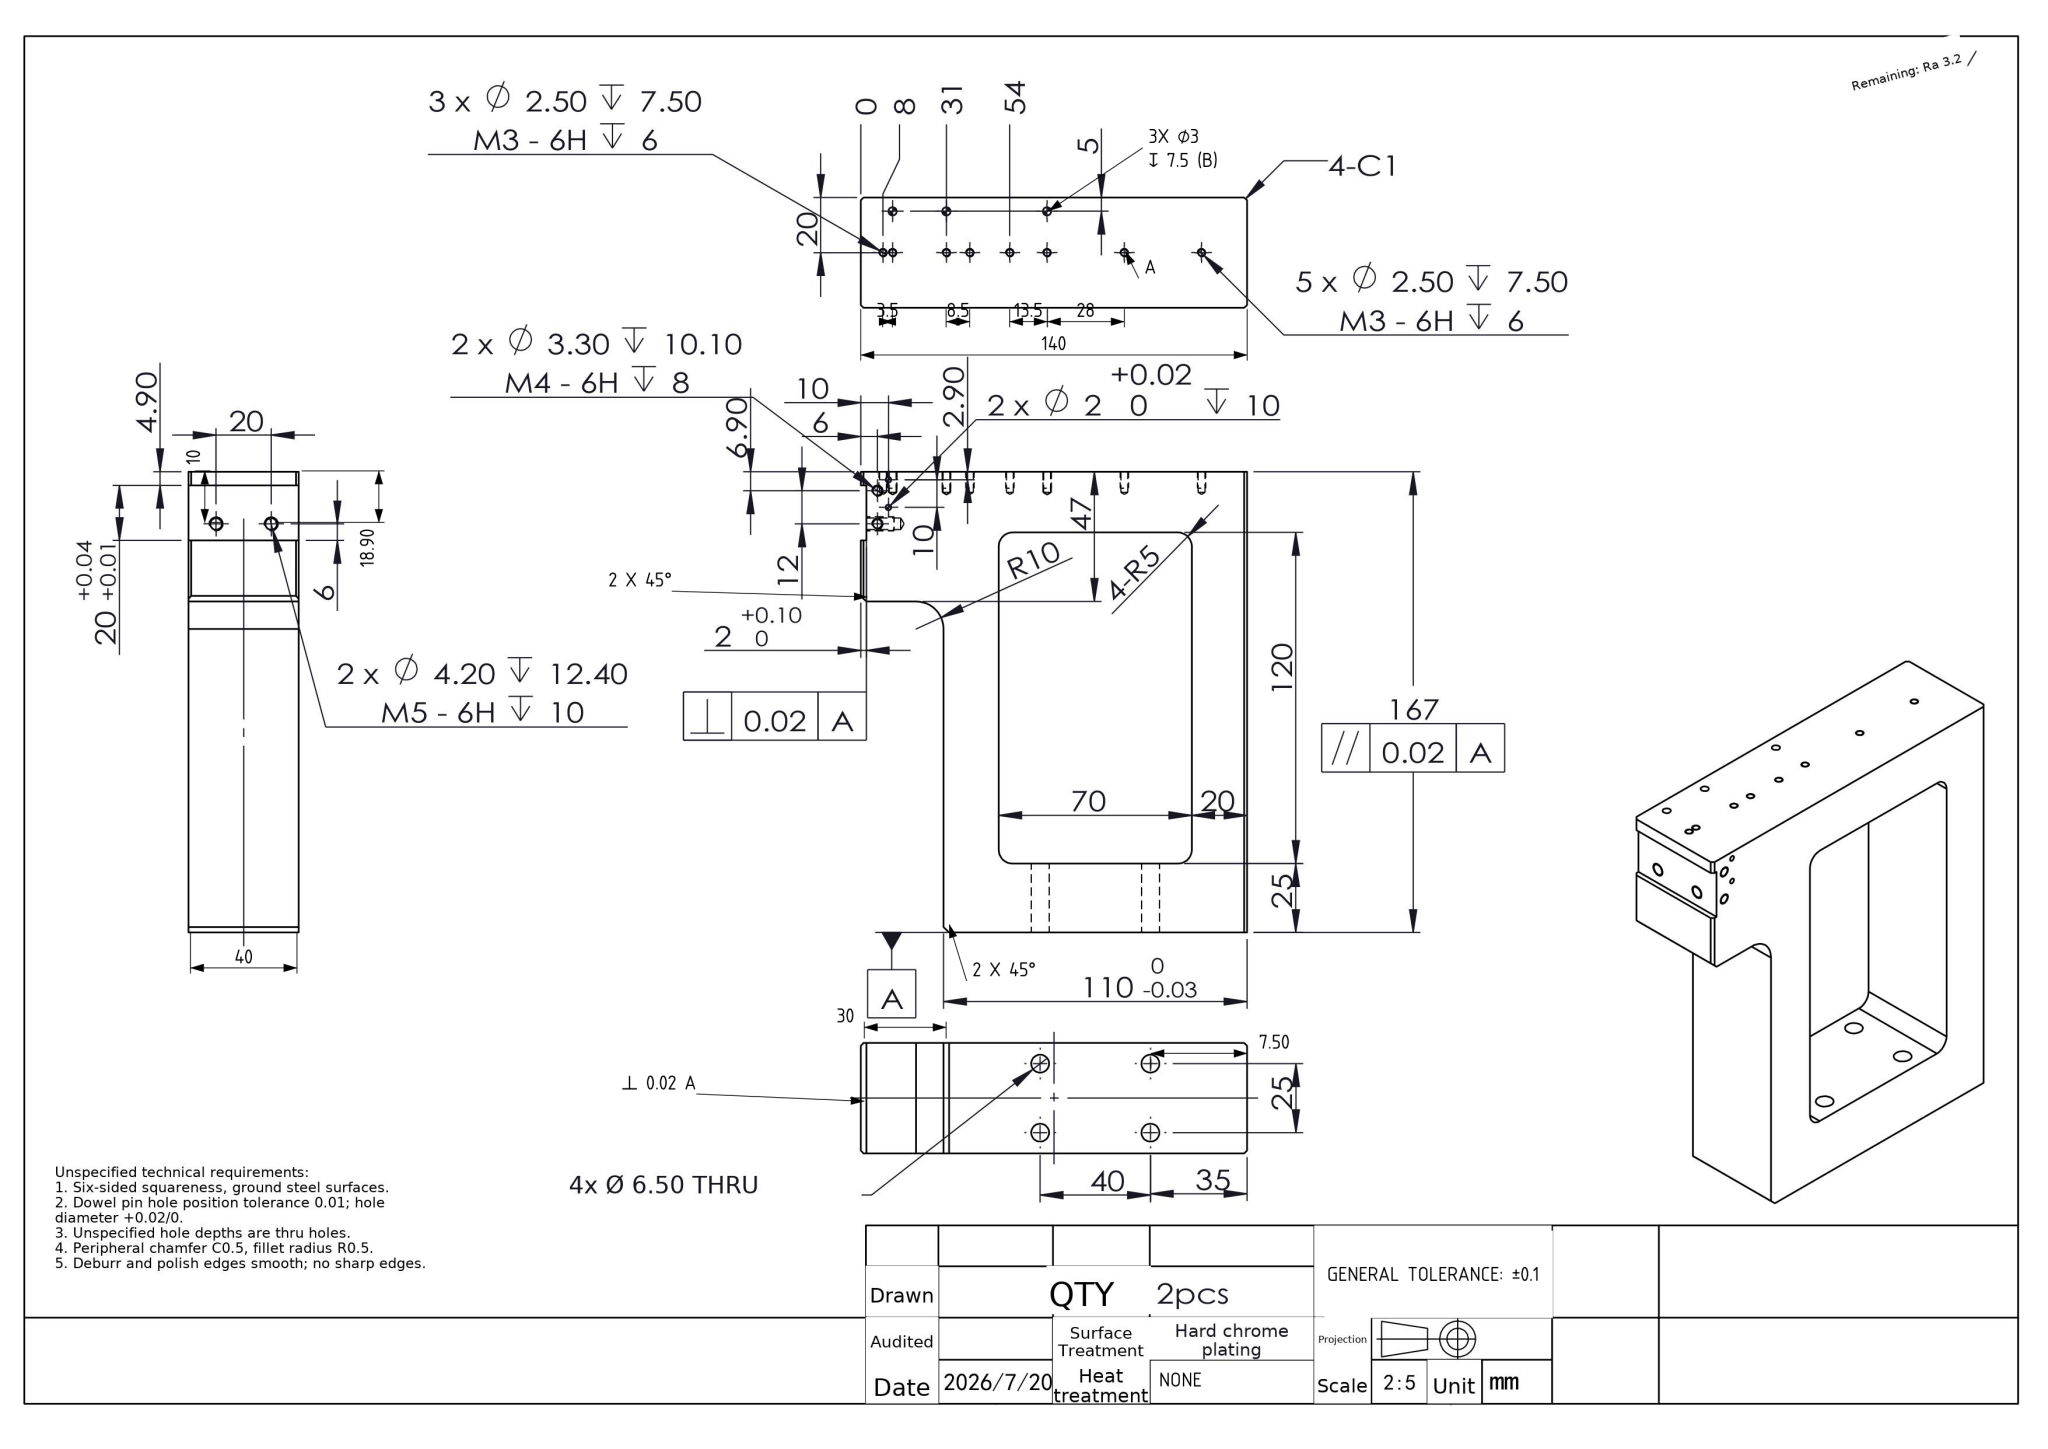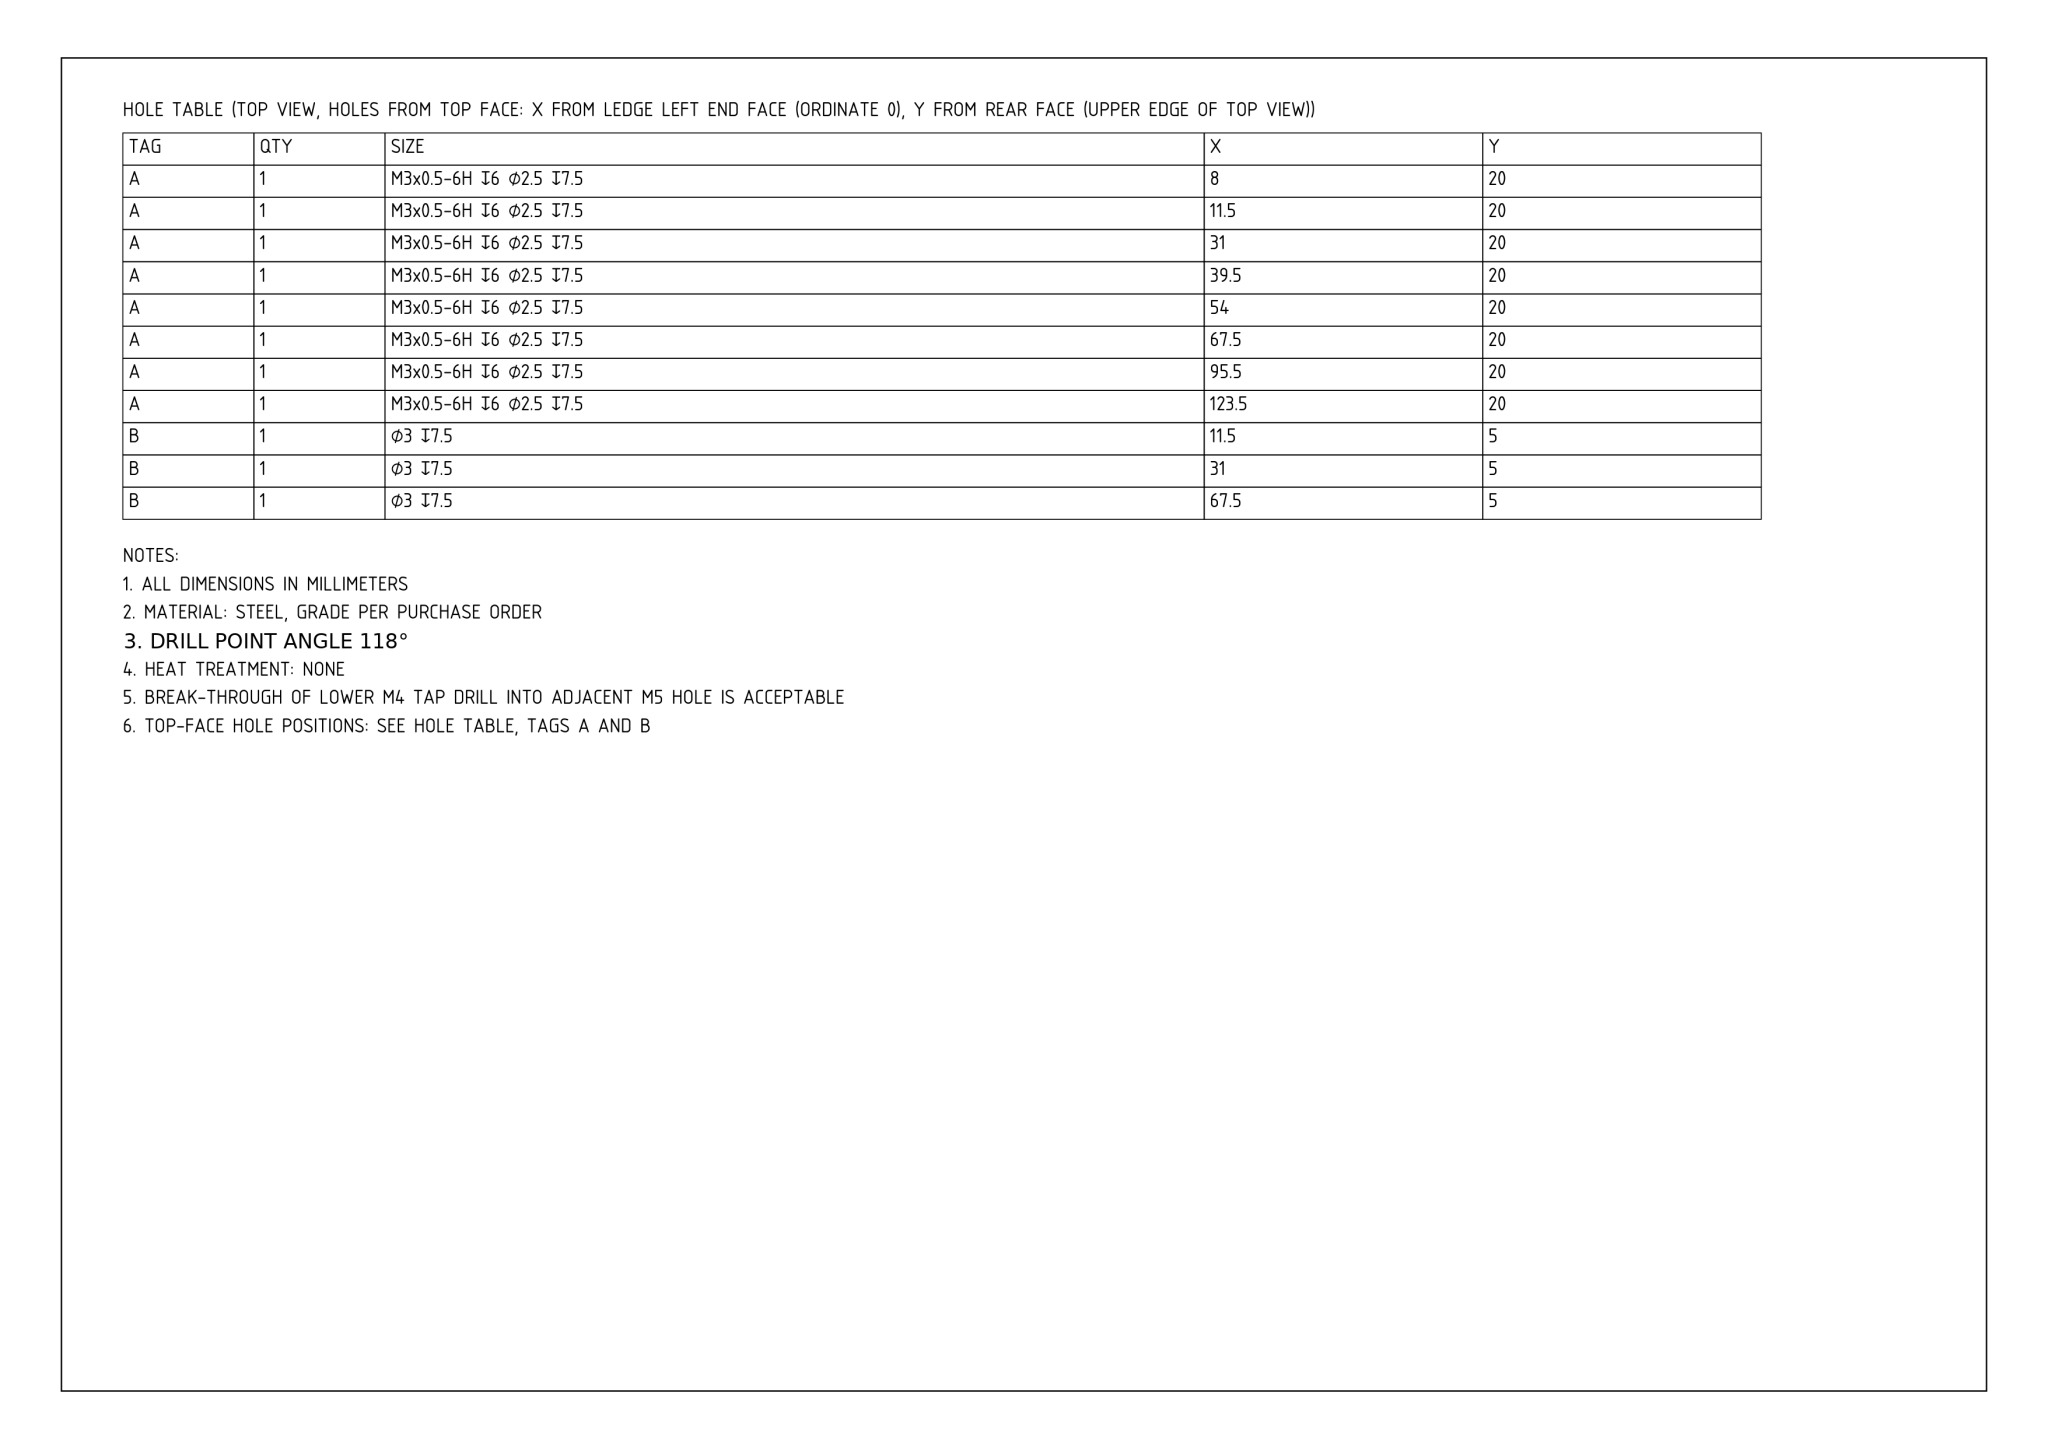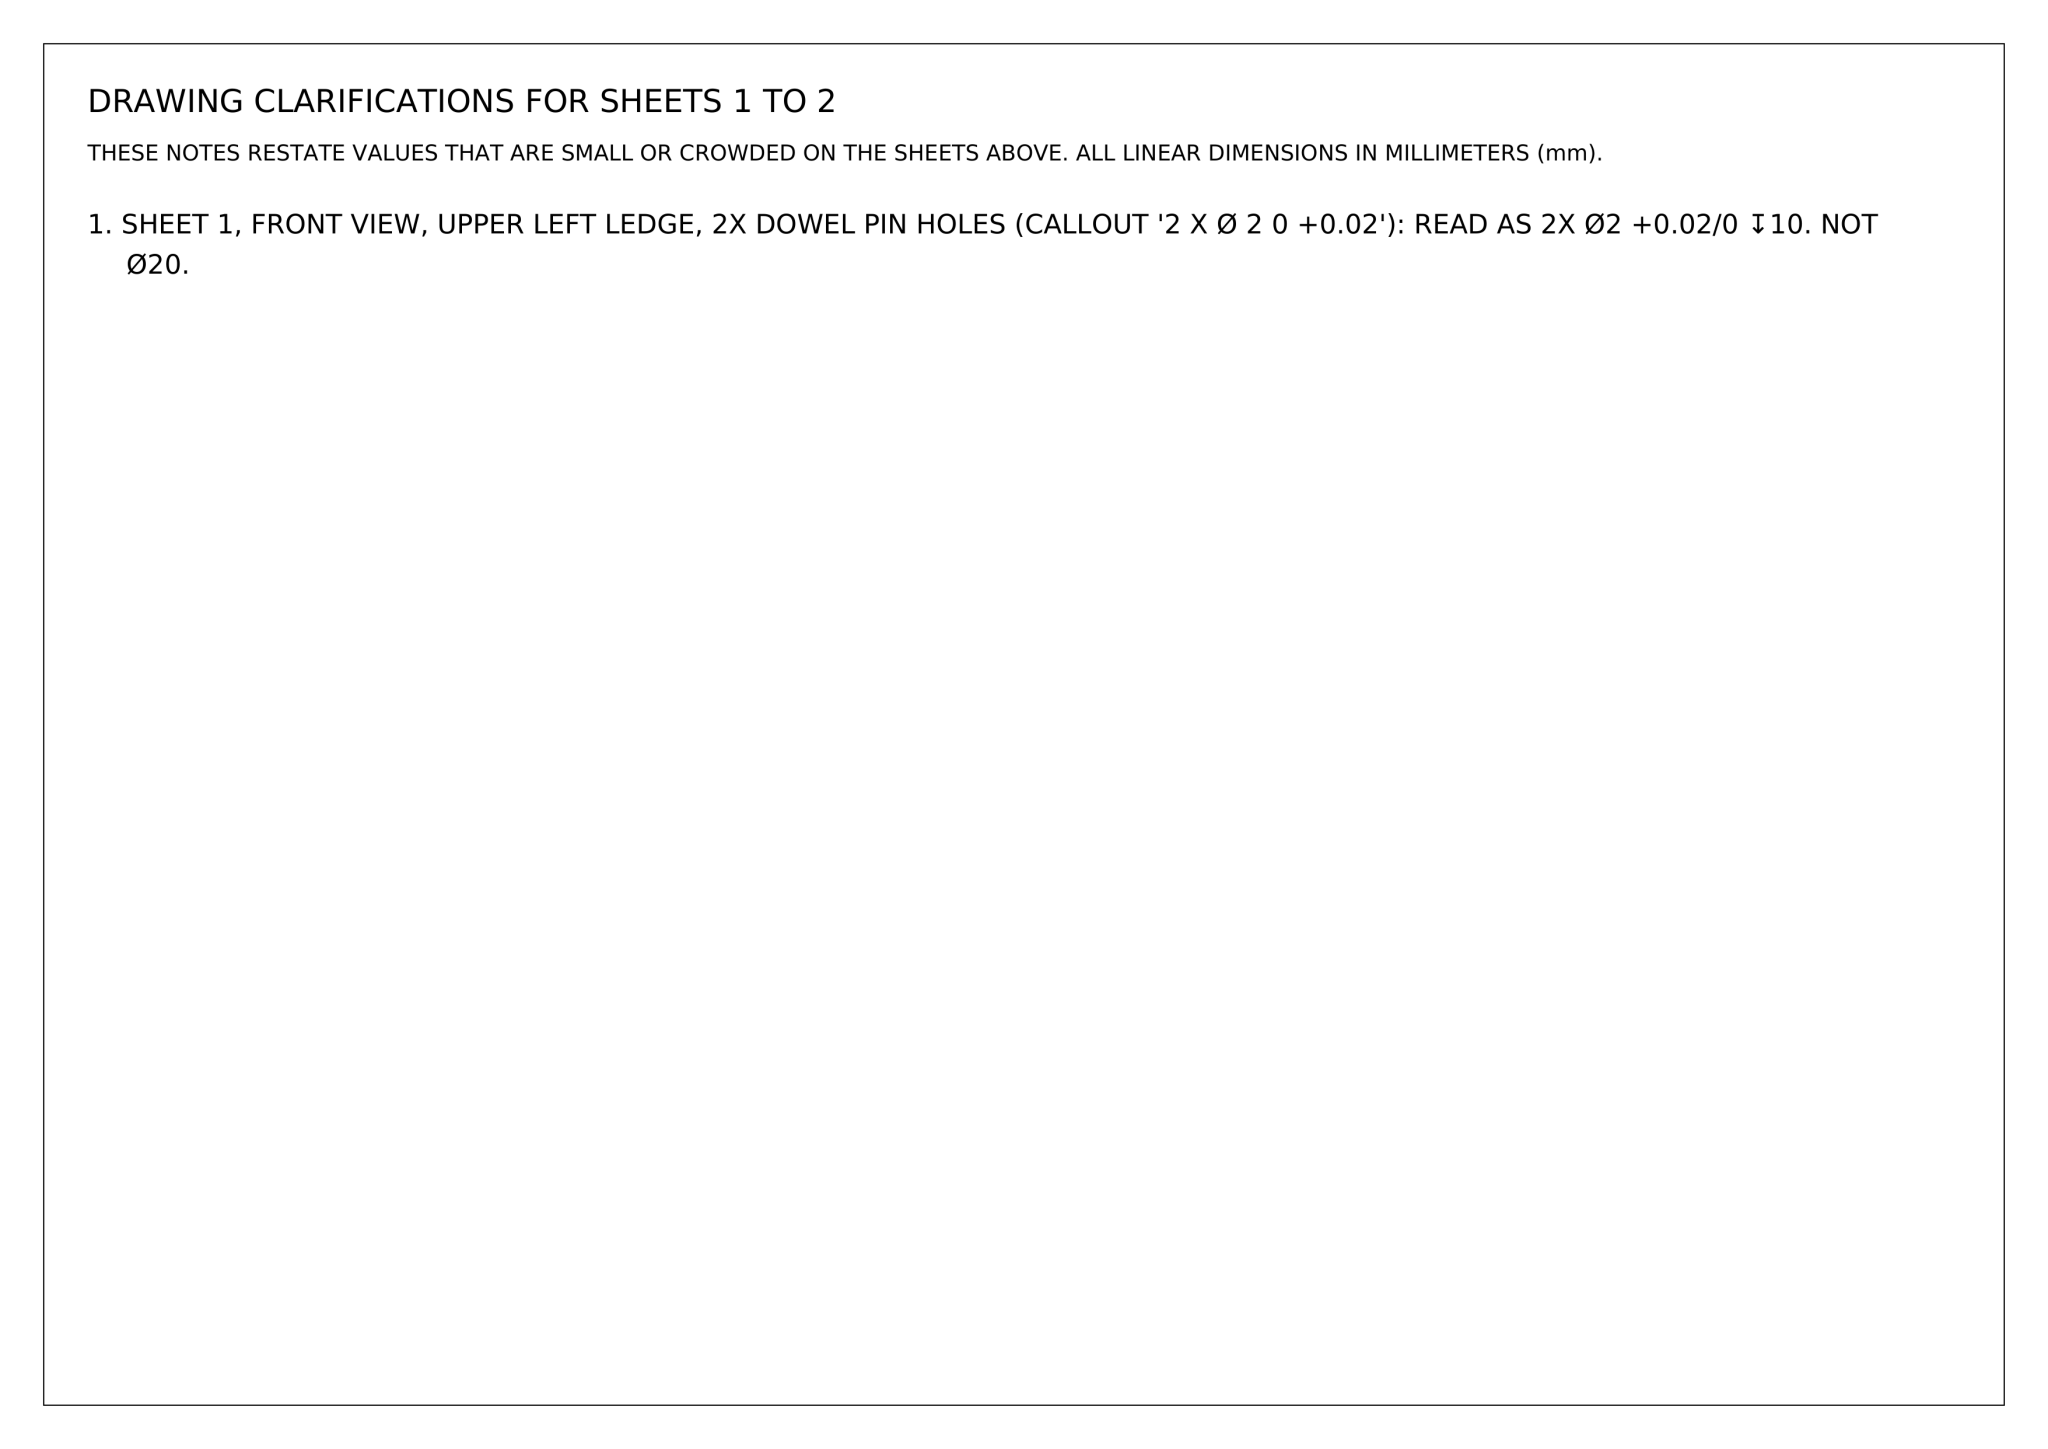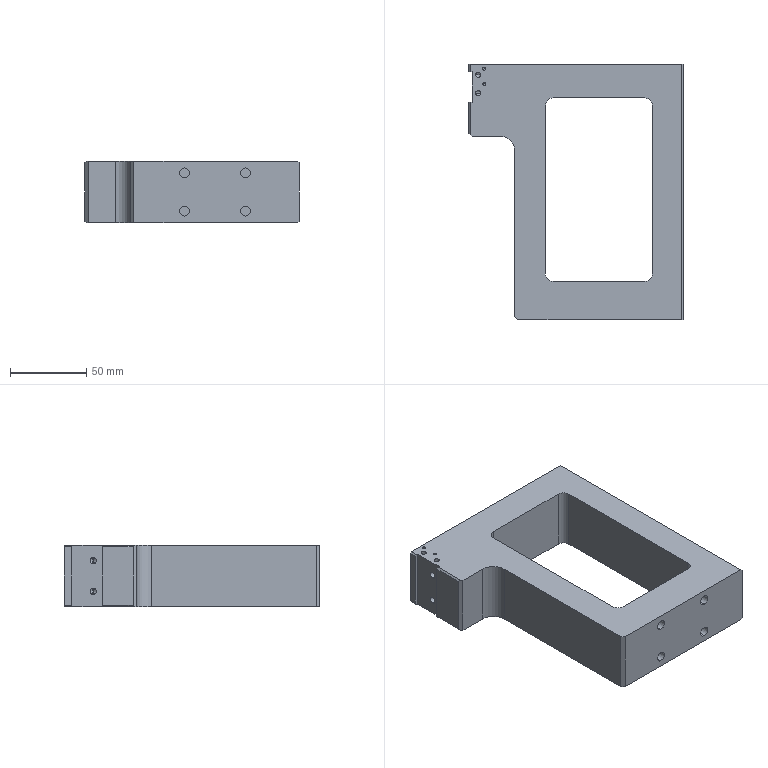Part | NX | mm | 1 solid | 103 faces | box 140 x 167 x 40 mm | volume 450599 mm3 | cylinder 47 | cone 32 | plane 24 | commonest cylinder face diameters 2.5 x16 6.5 x8 3 x6 2 x4 3.3 x4 4.2 x4 10 x4 20 x1